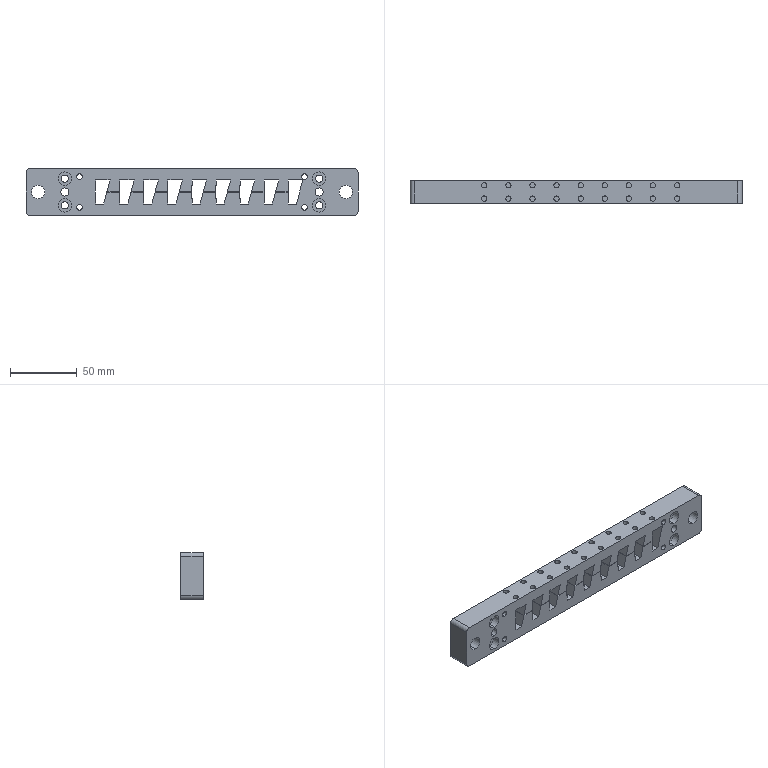Component | SolidWorks | 8TC-A15004-60-27A-1 | 1 solid | 204 faces | box 248 x 17 x 35 mm | volume 113846 mm3 | plane 114 | cylinder 90 | commonest cylinder face diameters 4 x36 3.3 x18 10 x12 5.3 x8 4.2 x8 6 x8 | material Cr12
build123d program:
from build123d import *

# Parameters (mm, degrees)
SKETCH1_W                                       = 248
SKETCH1_H                                       = 35
BOSS_EXTRUDE1_DEPTH                             = 8.5
SKETCH3_R                                       = 3
CUT_EXTRUDE2_DEPTH                              = 127.377
SKETCH4_R                                       = 5
CUT_EXTRUDE3_DEPTH                              = 127.377
CUT_EXTRUDE1_DEPTH                              = 127.377
SKETCH13_W                                      = 0.4
SKETCH13_H                                      = 9.5
CUT_EXTRUDE7_DEPTH                              = 127.377
LPATTERN1_COUNT                                 = 9
LPATTERN1_PITCH                                 = 18
M4_TAPPED_HOLE2_D                               = 4
M4_TAPPED_HOLE2_DEPTH                           = 8.5
LPATTERN2_COUNT                                 = 9
LPATTERN2_PITCH                                 = 18
SKETCH10_W                                      = 144.2
SKETCH10_H                                      = 0.2
CUT_EXTRUDE6_DEPTH                              = 127.377
M4_TAPPED_HOLE1_D                               = 3.3
M4_TAPPED_HOLE1_DEPTH                           = 8.5
FILLET1_R                                       = 3
LPATTERN3_COUNT                                 = 9
LPATTERN3_PITCH                                 = 18
M5_TAPPED_HOLE1_D                               = 4.2
M5_TAPPED_HOLE1_DEPTH                           = 19
M5_TAPPED_HOLE1_TIP                             = 1.262
M5_HEX_SOCKET_HEAD_CAP_SCREW_CBORE1_D           = 5.3
M5_HEX_SOCKET_HEAD_CAP_SCREW_CBORE1_CBORE_D     = 10
M5_HEX_SOCKET_HEAD_CAP_SCREW_CBORE1_CBORE_DEPTH = 5.4


with BuildPart() as part:
    # Sketch1 → Boss-Extrude1 (new, symmetric)
    with BuildSketch(Plane(origin=(0, 0, 0), x_dir=(1, 0, 0), z_dir=(0, 1, 0))):
        Rectangle(SKETCH1_W, SKETCH1_H)
    extrude(amount=BOSS_EXTRUDE1_DEPTH, both=True)

    # Sketch3 → Cut-Extrude2 (cut, through all)
    with BuildSketch(Plane.XZ.offset(8.5)):
        with Locations(Location((-95, 0, 0), (0, 0, 270))):
            Circle(SKETCH3_R)
        with Locations(Location((95, 0, 0), (0, 0, 90))):
            Circle(SKETCH3_R)
    extrude(amount=-CUT_EXTRUDE2_DEPTH, mode=Mode.SUBTRACT)

    # Sketch4 → Cut-Extrude3 (cut, through all)
    with BuildSketch(Plane.XZ.offset(8.5)):
        with Locations(Location((-115, 0, 0), (0, 0, 270))):
            Circle(SKETCH4_R)
        with Locations(Location((115, 0, 0), (0, 0, 90))):
            Circle(SKETCH4_R)
    extrude(amount=-CUT_EXTRUDE3_DEPTH, mode=Mode.SUBTRACT)

    # Sketch2 → Cut-Extrude1 (cut, through all)
    with BuildSketch(Plane.XZ.offset(8.5)):
        Polygon((-78, 9), (-72, 9), (-72, -9), (-82.823, -9), align=None)
    cut_extrude1 = extrude(amount=-CUT_EXTRUDE1_DEPTH, mode=Mode.SUBTRACT)

    # Sketch13 → Cut-Extrude7 (cut, through all)
    with BuildSketch(Plane.XZ.offset(8.5)):
        with Locations((-72, 0)):
            Rectangle(SKETCH13_W, SKETCH13_H)
    cut_extrude7 = extrude(amount=-CUT_EXTRUDE7_DEPTH, mode=Mode.SUBTRACT)

    # LPattern1: Cut-Extrude1, Cut-Extrude7 ×9
    with Locations(*[(i * LPATTERN1_PITCH, 0, 0) for i in range(1, LPATTERN1_COUNT)]):
        add(cut_extrude1, mode=Mode.SUBTRACT)
        add(cut_extrude7, mode=Mode.SUBTRACT)

    # M4 Tapped Hole2
    with Locations(Plane(origin=(0, 0, -17.5), x_dir=(-1, 0, 0), z_dir=(0, 0, -1))):
        with Locations((75.5, 5), (75.5, -5)):
            m4_tapped_hole2 = Hole(M4_TAPPED_HOLE2_D / 2, depth=M4_TAPPED_HOLE2_DEPTH)

    # LPattern2: M4 Tapped Hole2 ×9
    with Locations(*[(i * LPATTERN2_PITCH, 0, 0) for i in range(1, LPATTERN2_COUNT)]):
        add(m4_tapped_hole2, mode=Mode.SUBTRACT)

    # Sketch10 → Cut-Extrude6 (cut, through all)
    with BuildSketch(Plane.XZ.offset(8.5)):
        with Locations((0.1, 0)):
            Rectangle(SKETCH10_W, SKETCH10_H)
    extrude(amount=-CUT_EXTRUDE6_DEPTH, mode=Mode.SUBTRACT)

    # M4 Tapped Hole1
    with Locations(Plane.XY.offset(17.5)):
        with Locations((-75.5, 0)):
            m4_tapped_hole1 = Hole(M4_TAPPED_HOLE1_D / 2, depth=M4_TAPPED_HOLE1_DEPTH)

    # Fillet1
    fillet1_edges = [part.edges().sort_by_distance(p)[0] for p in [
        (124, 0, 17.5),
        (-124, 0, 17.5),
        (-124, 0, -17.5),
        (124, 0, -17.5),
    ]]
    fillet(fillet1_edges, radius=FILLET1_R)

    # LPattern3: M4 Tapped Hole1 ×9
    with Locations(*[(i * LPATTERN3_PITCH, 0, 0) for i in range(1, LPATTERN3_COUNT)]):
        add(m4_tapped_hole1, mode=Mode.SUBTRACT)

    # M5 Tapped Hole1
    with Locations(Plane(origin=(0, -8.5, 0), x_dir=(-1, 0, 0), z_dir=(0, -1, 0))):
        with Locations((84, -11.5), (84, 11.5), (-84, -11.5), (-84, 11.5)):
            Hole(M5_TAPPED_HOLE1_D / 2, depth=M5_TAPPED_HOLE1_DEPTH)
            with Locations((0, 0, -(M5_TAPPED_HOLE1_DEPTH + M5_TAPPED_HOLE1_TIP / 2))):  # 118° drill point
                Cone(0, M5_TAPPED_HOLE1_D / 2, M5_TAPPED_HOLE1_TIP, mode=Mode.SUBTRACT)

    # M5 Hex Socket Head Cap Screw CBORE1 (through all)
    with Locations(Plane(origin=(0, -8.5, 0), x_dir=(-1, 0, 0), z_dir=(0, -1, 0))):
        with Locations((-95, 10), (-95, -10), (95, -10), (95, 10)):
            CounterBoreHole(M5_HEX_SOCKET_HEAD_CAP_SCREW_CBORE1_D / 2, M5_HEX_SOCKET_HEAD_CAP_SCREW_CBORE1_CBORE_D / 2, M5_HEX_SOCKET_HEAD_CAP_SCREW_CBORE1_CBORE_DEPTH)


solid = part.part

# Placed as in the assembly
solid = solid.moved(Location((26.714, -68.5, 0), (-180, 0, 180)))